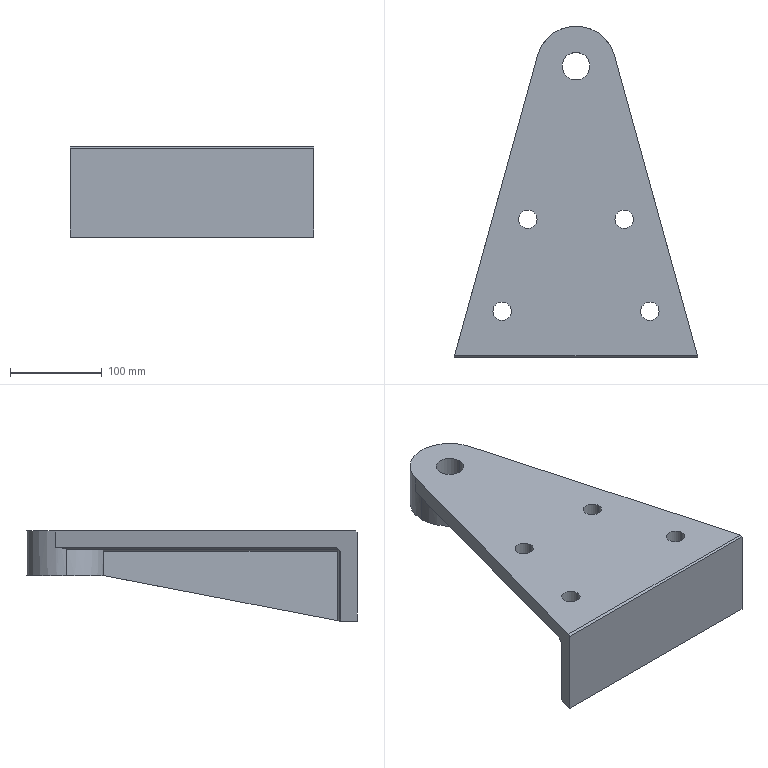Component | SolidWorks | SupportBase3-1 | 1 solid | 41 faces | volume 2111471 mm3 | plane 26 | cylinder 13 | spline 2 | commonest cylinder face diameters 20 x8 86.865 x3 30 x2 | material 45